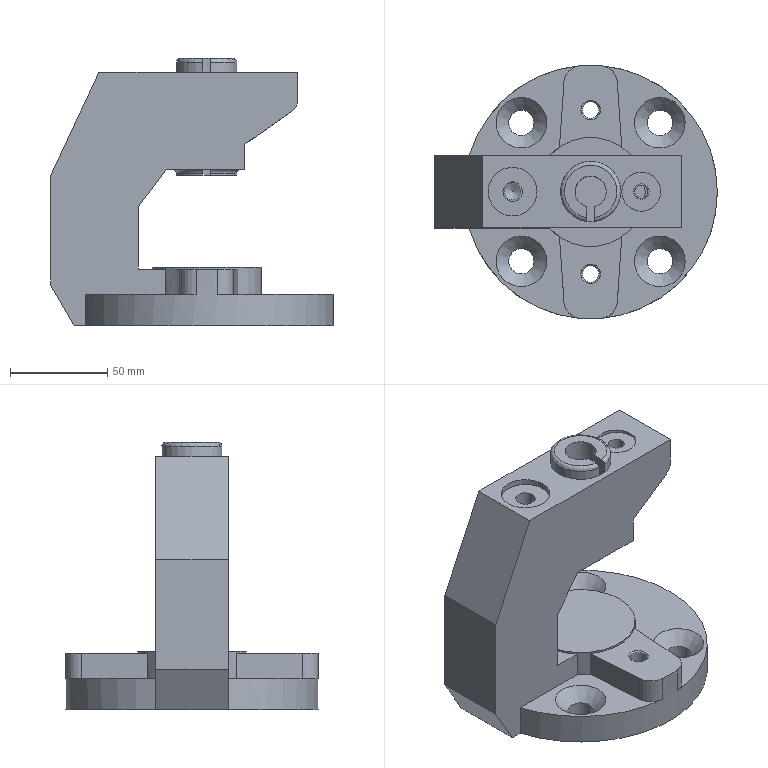Component | NX | BASE | 1 solid | 68 faces | volume 555574 mm3 | plane 32 | cylinder 24 | cone 9 | torus 2 | spline 1 | commonest cylinder face diameters 18 x4 13 x4 31 x3 8.5 x3 130 x1 56 x1 12 x1 16 x1